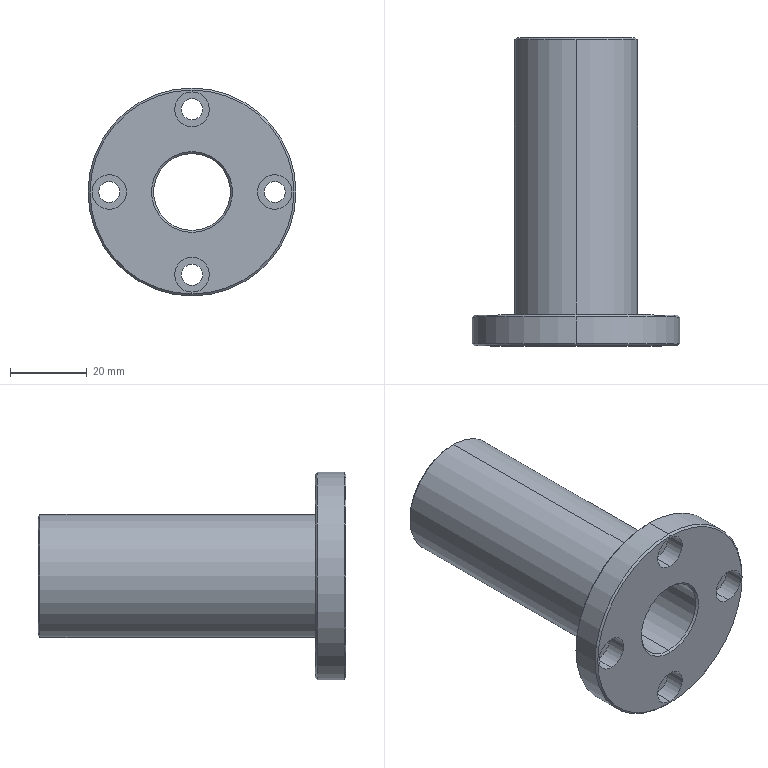Component | SolidWorks | FlangedLinearBearingLMF20L-1 | 1 solid | 39 faces | box 54 x 80 x 54 mm | volume 49451 mm3 | cylinder 22 | cone 10 | plane 7 | commonest cylinder face diameters 9 x8 5.5 x8 32 x2 54 x2 20 x2
STEP:
#1=CARTESIAN_POINT('',(-2.82,-0.6008,10.453));
#2=VERTEX_POINT('',#1);
#3=CARTESIAN_POINT('',(-2.82,-0.6008,10.807));
#4=VERTEX_POINT('',#3);
#5=CARTESIAN_POINT('',(-2.82,-0.6008,10.63));
#6=DIRECTION('',(0.,-1.,-0.));
#7=DIRECTION('',(0.,0.,1.));
#8=AXIS2_PLACEMENT_3D('',#5,#6,#7);
#9=CIRCLE('',#8,0.1772);
#10=EDGE_CURVE('',#2,#4,#9,.T.);
#11=ORIENTED_EDGE('',*,*,#10,.F.);
#12=CARTESIAN_POINT('',(-2.82,-0.8016,10.453));
#13=VERTEX_POINT('',#12);
#14=CARTESIAN_POINT('',(-2.82,-0.8016,10.453));
#15=DIRECTION('',(0.,-1.,-0.));
#16=VECTOR('',#15,39.37);
#17=LINE('',#14,#16);
#18=EDGE_CURVE('',#2,#13,#17,.T.);
#19=ORIENTED_EDGE('',*,*,#18,.T.);
#20=CARTESIAN_POINT('',(-2.82,-0.8016,10.807));
#21=VERTEX_POINT('',#20);
#22=CARTESIAN_POINT('',(-2.82,-0.8016,10.63));
#23=DIRECTION('',(0.,-1.,-0.));
#24=DIRECTION('',(0.,0.,1.));
#25=AXIS2_PLACEMENT_3D('',#22,#23,#24);
#26=CIRCLE('',#25,0.1772);
#27=EDGE_CURVE('',#13,#21,#26,.T.);
#28=ORIENTED_EDGE('',*,*,#27,.T.);
#29=CARTESIAN_POINT('',(-2.82,-0.8016,10.807));
#30=DIRECTION('',(0.,-1.,-0.));
#31=VECTOR('',#30,39.37);
#32=LINE('',#29,#31);
#33=EDGE_CURVE('',#4,#21,#32,.T.);
#34=ORIENTED_EDGE('',*,*,#33,.F.);
#35=EDGE_LOOP('',(#11,#19,#28,#34));
#36=FACE_OUTER_BOUND('',#35,.T.);
#37=CARTESIAN_POINT('',(-2.82,-0.8016,10.63));
#38=DIRECTION('',(0.,-1.,-0.));
#39=DIRECTION('',(0.,0.,1.));
#40=AXIS2_PLACEMENT_3D('',#37,#38,#39);
#41=CYLINDRICAL_SURFACE('',#40,0.1772);
#42=ADVANCED_FACE('',(#36),#41,.F.);
#43=CARTESIAN_POINT('',(-2.82,-0.4866,10.522));
#44=VERTEX_POINT('',#43);
#45=CARTESIAN_POINT('',(-2.82,-0.4866,10.738));
#46=VERTEX_POINT('',#45);
#47=CARTESIAN_POINT('',(-2.82,-0.4866,10.63));
#48=DIRECTION('',(0.,-1.,-0.));
#49=DIRECTION('',(0.,0.,1.));
#50=AXIS2_PLACEMENT_3D('',#47,#48,#49);
#51=CIRCLE('',#50,0.1083);
#52=EDGE_CURVE('',#44,#46,#51,.T.);
#53=ORIENTED_EDGE('',*,*,#52,.F.);
#54=CARTESIAN_POINT('',(-2.82,-0.6008,10.522));
#55=VERTEX_POINT('',#54);
#56=CARTESIAN_POINT('',(-2.82,-0.8016,10.522));
#57=DIRECTION('',(0.,-1.,-0.));
#58=VECTOR('',#57,39.37);
#59=LINE('',#56,#58);
#60=EDGE_CURVE('',#44,#55,#59,.T.);
#61=ORIENTED_EDGE('',*,*,#60,.T.);
#62=CARTESIAN_POINT('',(-2.82,-0.6008,10.738));
#63=VERTEX_POINT('',#62);
#64=CARTESIAN_POINT('',(-2.82,-0.6008,10.63));
#65=DIRECTION('',(0.,-1.,-0.));
#66=DIRECTION('',(0.,0.,1.));
#67=AXIS2_PLACEMENT_3D('',#64,#65,#66);
#68=CIRCLE('',#67,0.1083);
#69=EDGE_CURVE('',#55,#63,#68,.T.);
#70=ORIENTED_EDGE('',*,*,#69,.T.);
#71=CARTESIAN_POINT('',(-2.82,-0.8016,10.738));
#72=DIRECTION('',(0.,-1.,-0.));
#73=VECTOR('',#72,39.37);
#74=LINE('',#71,#73);
#75=EDGE_CURVE('',#46,#63,#74,.T.);
#76=ORIENTED_EDGE('',*,*,#75,.F.);
#77=EDGE_LOOP('',(#53,#61,#70,#76));
#78=FACE_OUTER_BOUND('',#77,.T.);
#79=CARTESIAN_POINT('',(-2.82,-0.8016,10.63));
#80=DIRECTION('',(0.,-1.,-0.));
#81=DIRECTION('',(0.,0.,1.));
#82=AXIS2_PLACEMENT_3D('',#79,#80,#81);
#83=CYLINDRICAL_SURFACE('',#82,0.1083);
#84=ADVANCED_FACE('',(#78),#83,.F.);
#85=CARTESIAN_POINT('',(-1.973,-0.6008,9.606));
#86=VERTEX_POINT('',#85);
#87=CARTESIAN_POINT('',(-1.973,-0.6008,9.961));
#88=VERTEX_POINT('',#87);
#89=CARTESIAN_POINT('',(-1.973,-0.6008,9.783));
#90=DIRECTION('',(0.,-1.,-0.));
#91=DIRECTION('',(0.,0.,1.));
#92=AXIS2_PLACEMENT_3D('',#89,#90,#91);
#93=CIRCLE('',#92,0.1772);
#94=EDGE_CURVE('',#86,#88,#93,.T.);
#95=ORIENTED_EDGE('',*,*,#94,.F.);
#96=CARTESIAN_POINT('',(-1.973,-0.8016,9.606));
#97=VERTEX_POINT('',#96);
#98=CARTESIAN_POINT('',(-1.973,-0.8016,9.606));
#99=DIRECTION('',(0.,-1.,-0.));
#100=VECTOR('',#99,39.37);
#101=LINE('',#98,#100);
#102=EDGE_CURVE('',#86,#97,#101,.T.);
#103=ORIENTED_EDGE('',*,*,#102,.T.);
#104=CARTESIAN_POINT('',(-1.973,-0.8016,9.961));
#105=VERTEX_POINT('',#104);
#106=CARTESIAN_POINT('',(-1.973,-0.8016,9.783));
#107=DIRECTION('',(0.,-1.,-0.));
#108=DIRECTION('',(0.,0.,1.));
#109=AXIS2_PLACEMENT_3D('',#106,#107,#108);
#110=CIRCLE('',#109,0.1772);
#111=EDGE_CURVE('',#97,#105,#110,.T.);
#112=ORIENTED_EDGE('',*,*,#111,.T.);
#113=CARTESIAN_POINT('',(-1.973,-0.8016,9.961));
#114=DIRECTION('',(0.,-1.,-0.));
#115=VECTOR('',#114,39.37);
#116=LINE('',#113,#115);
#117=EDGE_CURVE('',#88,#105,#116,.T.);
#118=ORIENTED_EDGE('',*,*,#117,.F.);
#119=EDGE_LOOP('',(#95,#103,#112,#118));
#120=FACE_OUTER_BOUND('',#119,.T.);
#121=CARTESIAN_POINT('',(-1.973,-0.8016,9.783));
#122=DIRECTION('',(0.,-1.,-0.));
#123=DIRECTION('',(0.,0.,1.));
#124=AXIS2_PLACEMENT_3D('',#121,#122,#123);
#125=CYLINDRICAL_SURFACE('',#124,0.1772);
#126=ADVANCED_FACE('',(#120),#125,.F.);
#127=CARTESIAN_POINT('',(-1.973,-0.4866,9.675));
#128=VERTEX_POINT('',#127);
#129=CARTESIAN_POINT('',(-1.973,-0.4866,9.892));
#130=VERTEX_POINT('',#129);
#131=CARTESIAN_POINT('',(-1.973,-0.4866,9.783));
#132=DIRECTION('',(0.,-1.,-0.));
#133=DIRECTION('',(0.,0.,1.));
#134=AXIS2_PLACEMENT_3D('',#131,#132,#133);
#135=CIRCLE('',#134,0.1083);
#136=EDGE_CURVE('',#128,#130,#135,.T.);
#137=ORIENTED_EDGE('',*,*,#136,.F.);
#138=CARTESIAN_POINT('',(-1.973,-0.6008,9.675));
#139=VERTEX_POINT('',#138);
#140=CARTESIAN_POINT('',(-1.973,-0.8016,9.675));
#141=DIRECTION('',(0.,-1.,-0.));
#142=VECTOR('',#141,39.37);
#143=LINE('',#140,#142);
#144=EDGE_CURVE('',#128,#139,#143,.T.);
#145=ORIENTED_EDGE('',*,*,#144,.T.);
#146=CARTESIAN_POINT('',(-1.973,-0.6008,9.892));
#147=VERTEX_POINT('',#146);
#148=CARTESIAN_POINT('',(-1.973,-0.6008,9.783));
#149=DIRECTION('',(0.,-1.,-0.));
#150=DIRECTION('',(0.,0.,1.));
#151=AXIS2_PLACEMENT_3D('',#148,#149,#150);
#152=CIRCLE('',#151,0.1083);
#153=EDGE_CURVE('',#139,#147,#152,.T.);
#154=ORIENTED_EDGE('',*,*,#153,.T.);
#155=CARTESIAN_POINT('',(-1.973,-0.8016,9.892));
#156=DIRECTION('',(0.,-1.,-0.));
#157=VECTOR('',#156,39.37);
#158=LINE('',#155,#157);
#159=EDGE_CURVE('',#130,#147,#158,.T.);
#160=ORIENTED_EDGE('',*,*,#159,.F.);
#161=EDGE_LOOP('',(#137,#145,#154,#160));
#162=FACE_OUTER_BOUND('',#161,.T.);
#163=CARTESIAN_POINT('',(-1.973,-0.8016,9.783));
#164=DIRECTION('',(0.,-1.,-0.));
#165=DIRECTION('',(0.,0.,1.));
#166=AXIS2_PLACEMENT_3D('',#163,#164,#165);
#167=CYLINDRICAL_SURFACE('',#166,0.1083);
#168=ADVANCED_FACE('',(#162),#167,.F.);
#169=CARTESIAN_POINT('',(-1.973,-0.6008,11.299));
#170=VERTEX_POINT('',#169);
#171=CARTESIAN_POINT('',(-1.973,-0.6008,11.654));
#172=VERTEX_POINT('',#171);
#173=CARTESIAN_POINT('',(-1.973,-0.6008,11.476));
#174=DIRECTION('',(0.,-1.,-0.));
#175=DIRECTION('',(0.,0.,1.));
#176=AXIS2_PLACEMENT_3D('',#173,#174,#175);
#177=CIRCLE('',#176,0.1772);
#178=EDGE_CURVE('',#170,#172,#177,.T.);
#179=ORIENTED_EDGE('',*,*,#178,.F.);
#180=CARTESIAN_POINT('',(-1.973,-0.8016,11.299));
#181=VERTEX_POINT('',#180);
#182=CARTESIAN_POINT('',(-1.973,-0.8016,11.299));
#183=DIRECTION('',(0.,-1.,-0.));
#184=VECTOR('',#183,39.37);
#185=LINE('',#182,#184);
#186=EDGE_CURVE('',#170,#181,#185,.T.);
#187=ORIENTED_EDGE('',*,*,#186,.T.);
#188=CARTESIAN_POINT('',(-1.973,-0.8016,11.654));
#189=VERTEX_POINT('',#188);
#190=CARTESIAN_POINT('',(-1.973,-0.8016,11.476));
#191=DIRECTION('',(0.,-1.,-0.));
#192=DIRECTION('',(0.,0.,1.));
#193=AXIS2_PLACEMENT_3D('',#190,#191,#192);
#194=CIRCLE('',#193,0.1772);
#195=EDGE_CURVE('',#181,#189,#194,.T.);
#196=ORIENTED_EDGE('',*,*,#195,.T.);
#197=CARTESIAN_POINT('',(-1.973,-0.8016,11.654));
#198=DIRECTION('',(0.,-1.,-0.));
#199=VECTOR('',#198,39.37);
#200=LINE('',#197,#199);
#201=EDGE_CURVE('',#172,#189,#200,.T.);
#202=ORIENTED_EDGE('',*,*,#201,.F.);
#203=EDGE_LOOP('',(#179,#187,#196,#202));
#204=FACE_OUTER_BOUND('',#203,.T.);
#205=CARTESIAN_POINT('',(-1.973,-0.8016,11.476));
#206=DIRECTION('',(0.,-1.,-0.));
#207=DIRECTION('',(0.,0.,1.));
#208=AXIS2_PLACEMENT_3D('',#205,#206,#207);
#209=CYLINDRICAL_SURFACE('',#208,0.1772);
#210=ADVANCED_FACE('',(#204),#209,.F.);
#211=CARTESIAN_POINT('',(-1.973,-0.4866,11.368));
#212=VERTEX_POINT('',#211);
#213=CARTESIAN_POINT('',(-1.973,-0.4866,11.585));
#214=VERTEX_POINT('',#213);
#215=CARTESIAN_POINT('',(-1.973,-0.4866,11.476));
#216=DIRECTION('',(0.,-1.,-0.));
#217=DIRECTION('',(0.,0.,1.));
#218=AXIS2_PLACEMENT_3D('',#215,#216,#217);
#219=CIRCLE('',#218,0.1083);
#220=EDGE_CURVE('',#212,#214,#219,.T.);
#221=ORIENTED_EDGE('',*,*,#220,.F.);
#222=CARTESIAN_POINT('',(-1.973,-0.6008,11.368));
#223=VERTEX_POINT('',#222);
#224=CARTESIAN_POINT('',(-1.973,-0.8016,11.368));
#225=DIRECTION('',(0.,-1.,-0.));
#226=VECTOR('',#225,39.37);
#227=LINE('',#224,#226);
#228=EDGE_CURVE('',#212,#223,#227,.T.);
#229=ORIENTED_EDGE('',*,*,#228,.T.);
#230=CARTESIAN_POINT('',(-1.973,-0.6008,11.585));
#231=VERTEX_POINT('',#230);
#232=CARTESIAN_POINT('',(-1.973,-0.6008,11.476));
#233=DIRECTION('',(0.,-1.,-0.));
#234=DIRECTION('',(0.,0.,1.));
#235=AXIS2_PLACEMENT_3D('',#232,#233,#234);
#236=CIRCLE('',#235,0.1083);
#237=EDGE_CURVE('',#223,#231,#236,.T.);
#238=ORIENTED_EDGE('',*,*,#237,.T.);
#239=CARTESIAN_POINT('',(-1.973,-0.8016,11.585));
#240=DIRECTION('',(0.,-1.,-0.));
#241=VECTOR('',#240,39.37);
#242=LINE('',#239,#241);
#243=EDGE_CURVE('',#214,#231,#242,.T.);
#244=ORIENTED_EDGE('',*,*,#243,.F.);
#245=EDGE_LOOP('',(#221,#229,#238,#244));
#246=FACE_OUTER_BOUND('',#245,.T.);
#247=CARTESIAN_POINT('',(-1.973,-0.8016,11.476));
#248=DIRECTION('',(0.,-1.,-0.));
#249=DIRECTION('',(0.,0.,1.));
#250=AXIS2_PLACEMENT_3D('',#247,#248,#249);
#251=CYLINDRICAL_SURFACE('',#250,0.1083);
#252=ADVANCED_FACE('',(#246),#251,.F.);
#253=CARTESIAN_POINT('',(-1.127,-0.6008,10.453));
#254=VERTEX_POINT('',#253);
#255=CARTESIAN_POINT('',(-1.127,-0.6008,10.807));
#256=VERTEX_POINT('',#255);
#257=CARTESIAN_POINT('',(-1.127,-0.6008,10.63));
#258=DIRECTION('',(0.,-1.,-0.));
#259=DIRECTION('',(0.,0.,1.));
#260=AXIS2_PLACEMENT_3D('',#257,#258,#259);
#261=CIRCLE('',#260,0.1772);
#262=EDGE_CURVE('',#254,#256,#261,.T.);
#263=ORIENTED_EDGE('',*,*,#262,.F.);
#264=CARTESIAN_POINT('',(-1.127,-0.8016,10.453));
#265=VERTEX_POINT('',#264);
#266=CARTESIAN_POINT('',(-1.127,-0.8016,10.453));
#267=DIRECTION('',(0.,-1.,-0.));
#268=VECTOR('',#267,39.37);
#269=LINE('',#266,#268);
#270=EDGE_CURVE('',#254,#265,#269,.T.);
#271=ORIENTED_EDGE('',*,*,#270,.T.);
#272=CARTESIAN_POINT('',(-1.127,-0.8016,10.807));
#273=VERTEX_POINT('',#272);
#274=CARTESIAN_POINT('',(-1.127,-0.8016,10.63));
#275=DIRECTION('',(0.,-1.,-0.));
#276=DIRECTION('',(0.,0.,1.));
#277=AXIS2_PLACEMENT_3D('',#274,#275,#276);
#278=CIRCLE('',#277,0.1772);
#279=EDGE_CURVE('',#265,#273,#278,.T.);
#280=ORIENTED_EDGE('',*,*,#279,.T.);
#281=CARTESIAN_POINT('',(-1.127,-0.8016,10.807));
#282=DIRECTION('',(0.,-1.,-0.));
#283=VECTOR('',#282,39.37);
#284=LINE('',#281,#283);
#285=EDGE_CURVE('',#256,#273,#284,.T.);
#286=ORIENTED_EDGE('',*,*,#285,.F.);
#287=EDGE_LOOP('',(#263,#271,#280,#286));
#288=FACE_OUTER_BOUND('',#287,.T.);
#289=CARTESIAN_POINT('',(-1.127,-0.8016,10.63));
#290=DIRECTION('',(0.,-1.,-0.));
#291=DIRECTION('',(0.,0.,1.));
#292=AXIS2_PLACEMENT_3D('',#289,#290,#291);
#293=CYLINDRICAL_SURFACE('',#292,0.1772);
#294=ADVANCED_FACE('',(#288),#293,.F.);
#295=CARTESIAN_POINT('',(-1.127,-0.4866,10.522));
#296=VERTEX_POINT('',#295);
#297=CARTESIAN_POINT('',(-1.127,-0.4866,10.738));
#298=VERTEX_POINT('',#297);
#299=CARTESIAN_POINT('',(-1.127,-0.4866,10.63));
#300=DIRECTION('',(0.,-1.,-0.));
#301=DIRECTION('',(0.,0.,1.));
#302=AXIS2_PLACEMENT_3D('',#299,#300,#301);
#303=CIRCLE('',#302,0.1083);
#304=EDGE_CURVE('',#296,#298,#303,.T.);
#305=ORIENTED_EDGE('',*,*,#304,.F.);
#306=CARTESIAN_POINT('',(-1.127,-0.6008,10.522));
#307=VERTEX_POINT('',#306);
#308=CARTESIAN_POINT('',(-1.127,-0.8016,10.522));
#309=DIRECTION('',(0.,-1.,-0.));
#310=VECTOR('',#309,39.37);
#311=LINE('',#308,#310);
#312=EDGE_CURVE('',#296,#307,#311,.T.);
#313=ORIENTED_EDGE('',*,*,#312,.T.);
#314=CARTESIAN_POINT('',(-1.127,-0.6008,10.738));
#315=VERTEX_POINT('',#314);
#316=CARTESIAN_POINT('',(-1.127,-0.6008,10.63));
#317=DIRECTION('',(0.,-1.,-0.));
#318=DIRECTION('',(0.,0.,1.));
#319=AXIS2_PLACEMENT_3D('',#316,#317,#318);
#320=CIRCLE('',#319,0.1083);
#321=EDGE_CURVE('',#307,#315,#320,.T.);
#322=ORIENTED_EDGE('',*,*,#321,.T.);
#323=CARTESIAN_POINT('',(-1.127,-0.8016,10.738));
#324=DIRECTION('',(0.,-1.,-0.));
#325=VECTOR('',#324,39.37);
#326=LINE('',#323,#325);
#327=EDGE_CURVE('',#298,#315,#326,.T.);
#328=ORIENTED_EDGE('',*,*,#327,.F.);
#329=EDGE_LOOP('',(#305,#313,#322,#328));
#330=FACE_OUTER_BOUND('',#329,.T.);
#331=CARTESIAN_POINT('',(-1.127,-0.8016,10.63));
#332=DIRECTION('',(0.,-1.,-0.));
#333=DIRECTION('',(0.,0.,1.));
#334=AXIS2_PLACEMENT_3D('',#331,#332,#333);
#335=CYLINDRICAL_SURFACE('',#334,0.1083);
#336=ADVANCED_FACE('',(#330),#335,.F.);
#337=CARTESIAN_POINT('',(-1.973,-0.8016,11.673));
#338=VERTEX_POINT('',#337);
#339=CARTESIAN_POINT('',(-1.973,-0.8016,9.587));
#340=VERTEX_POINT('',#339);
#341=CARTESIAN_POINT('',(-1.973,-0.8016,10.63));
#342=DIRECTION('',(0.,-1.,-0.));
#343=DIRECTION('',(-0.,0.,-1.));
#344=AXIS2_PLACEMENT_3D('',#341,#342,#343);
#345=CIRCLE('',#344,1.043);
#346=EDGE_CURVE('',#338,#340,#345,.T.);
#347=ORIENTED_EDGE('',*,*,#346,.F.);
#348=CARTESIAN_POINT('',(-1.973,-0.7819,11.693));
#349=VERTEX_POINT('',#348);
#350=CARTESIAN_POINT('',(-1.973,-0.8016,11.673));
#351=DIRECTION('',(0.,0.7071,0.7071));
#352=VECTOR('',#351,39.37);
#353=LINE('',#350,#352);
#354=EDGE_CURVE('',#338,#349,#353,.T.);
#355=ORIENTED_EDGE('',*,*,#354,.T.);
#356=CARTESIAN_POINT('',(-1.973,-0.7819,9.567));
#357=VERTEX_POINT('',#356);
#358=CARTESIAN_POINT('',(-1.973,-0.7819,10.63));
#359=DIRECTION('',(-0.,1.,0.));
#360=DIRECTION('',(-0.,0.,-1.));
#361=AXIS2_PLACEMENT_3D('',#358,#359,#360);
#362=CIRCLE('',#361,1.063);
#363=EDGE_CURVE('',#357,#349,#362,.T.);
#364=ORIENTED_EDGE('',*,*,#363,.F.);
#365=CARTESIAN_POINT('',(-1.973,-0.8016,9.587));
#366=DIRECTION('',(-0.,0.7071,-0.7071));
#367=VECTOR('',#366,39.37);
#368=LINE('',#365,#367);
#369=EDGE_CURVE('',#340,#357,#368,.T.);
#370=ORIENTED_EDGE('',*,*,#369,.F.);
#371=EDGE_LOOP('',(#347,#355,#364,#370));
#372=FACE_OUTER_BOUND('',#371,.T.);
#373=CARTESIAN_POINT('',(-1.973,-0.8016,10.63));
#374=DIRECTION('',(-0.,1.,0.));
#375=DIRECTION('',(-0.,0.,-1.));
#376=AXIS2_PLACEMENT_3D('',#373,#374,#375);
#377=CONICAL_SURFACE('',#376,1.043,0.7854);
#378=ADVANCED_FACE('',(#372),#377,.T.);
#379=CARTESIAN_POINT('',(-1.973,-0.4866,9.587));
#380=VERTEX_POINT('',#379);
#381=CARTESIAN_POINT('',(-1.973,-0.4866,11.673));
#382=VERTEX_POINT('',#381);
#383=CARTESIAN_POINT('',(-1.973,-0.4866,10.63));
#384=DIRECTION('',(-0.,1.,0.));
#385=DIRECTION('',(0.,-0.,1.));
#386=AXIS2_PLACEMENT_3D('',#383,#384,#385);
#387=CIRCLE('',#386,1.043);
#388=EDGE_CURVE('',#380,#382,#387,.T.);
#389=ORIENTED_EDGE('',*,*,#388,.F.);
#390=CARTESIAN_POINT('',(-1.973,-0.5063,9.567));
#391=VERTEX_POINT('',#390);
#392=CARTESIAN_POINT('',(-1.973,-0.5063,9.567));
#393=DIRECTION('',(-0.,-0.7071,-0.7071));
#394=VECTOR('',#393,39.37);
#395=LINE('',#392,#394);
#396=EDGE_CURVE('',#380,#391,#395,.T.);
#397=ORIENTED_EDGE('',*,*,#396,.T.);
#398=CARTESIAN_POINT('',(-1.973,-0.5063,11.693));
#399=VERTEX_POINT('',#398);
#400=CARTESIAN_POINT('',(-1.973,-0.5063,10.63));
#401=DIRECTION('',(0.,-1.,-0.));
#402=DIRECTION('',(0.,-0.,1.));
#403=AXIS2_PLACEMENT_3D('',#400,#401,#402);
#404=CIRCLE('',#403,1.063);
#405=EDGE_CURVE('',#399,#391,#404,.T.);
#406=ORIENTED_EDGE('',*,*,#405,.F.);
#407=CARTESIAN_POINT('',(-1.973,-0.5063,11.693));
#408=DIRECTION('',(0.,-0.7071,0.7071));
#409=VECTOR('',#408,39.37);
#410=LINE('',#407,#409);
#411=EDGE_CURVE('',#382,#399,#410,.T.);
#412=ORIENTED_EDGE('',*,*,#411,.F.);
#413=EDGE_LOOP('',(#389,#397,#406,#412));
#414=FACE_OUTER_BOUND('',#413,.T.);
#415=CARTESIAN_POINT('',(-1.973,-0.5063,10.63));
#416=DIRECTION('',(0.,-1.,-0.));
#417=DIRECTION('',(0.,-0.,1.));
#418=AXIS2_PLACEMENT_3D('',#415,#416,#417);
#419=CONICAL_SURFACE('',#418,1.063,0.7854);
#420=ADVANCED_FACE('',(#414),#419,.T.);
#421=CARTESIAN_POINT('',(-1.973,-0.7819,10.236));
#422=VERTEX_POINT('',#421);
#423=CARTESIAN_POINT('',(-1.973,-0.7819,11.024));
#424=VERTEX_POINT('',#423);
#425=CARTESIAN_POINT('',(-1.973,-0.7819,10.63));
#426=DIRECTION('',(0.,-1.,-0.));
#427=DIRECTION('',(-0.,0.,-1.));
#428=AXIS2_PLACEMENT_3D('',#425,#426,#427);
#429=CIRCLE('',#428,0.3937);
#430=EDGE_CURVE('',#422,#424,#429,.T.);
#431=ORIENTED_EDGE('',*,*,#430,.F.);
#432=CARTESIAN_POINT('',(-1.973,-0.8016,10.217));
#433=VERTEX_POINT('',#432);
#434=CARTESIAN_POINT('',(-1.973,-0.7819,10.236));
#435=DIRECTION('',(-0.,-0.7071,-0.7071));
#436=VECTOR('',#435,39.37);
#437=LINE('',#434,#436);
#438=EDGE_CURVE('',#422,#433,#437,.T.);
#439=ORIENTED_EDGE('',*,*,#438,.T.);
#440=CARTESIAN_POINT('',(-1.973,-0.8016,11.043));
#441=VERTEX_POINT('',#440);
#442=CARTESIAN_POINT('',(-1.973,-0.8016,10.63));
#443=DIRECTION('',(-0.,1.,0.));
#444=DIRECTION('',(-0.,0.,-1.));
#445=AXIS2_PLACEMENT_3D('',#442,#443,#444);
#446=CIRCLE('',#445,0.4134);
#447=EDGE_CURVE('',#441,#433,#446,.T.);
#448=ORIENTED_EDGE('',*,*,#447,.F.);
#449=CARTESIAN_POINT('',(-1.973,-0.7819,11.024));
#450=DIRECTION('',(0.,-0.7071,0.7071));
#451=VECTOR('',#450,39.37);
#452=LINE('',#449,#451);
#453=EDGE_CURVE('',#424,#441,#452,.T.);
#454=ORIENTED_EDGE('',*,*,#453,.F.);
#455=EDGE_LOOP('',(#431,#439,#448,#454));
#456=FACE_OUTER_BOUND('',#455,.T.);
#457=CARTESIAN_POINT('',(-1.973,-0.7819,10.63));
#458=DIRECTION('',(0.,-1.,-0.));
#459=DIRECTION('',(0.,0.,1.));
#460=AXIS2_PLACEMENT_3D('',#457,#458,#459);
#461=CONICAL_SURFACE('',#460,0.3937,0.7854);
#462=ADVANCED_FACE('',(#456),#461,.F.);
#463=CARTESIAN_POINT('',(-1.973,2.348,10.02));
#464=VERTEX_POINT('',#463);
#465=CARTESIAN_POINT('',(-1.973,2.348,11.24));
#466=VERTEX_POINT('',#465);
#467=CARTESIAN_POINT('',(-1.973,2.348,10.63));
#468=DIRECTION('',(-0.,1.,0.));
#469=DIRECTION('',(0.,0.,1.));
#470=AXIS2_PLACEMENT_3D('',#467,#468,#469);
#471=CIRCLE('',#470,0.6102);
#472=EDGE_CURVE('',#464,#466,#471,.T.);
#473=ORIENTED_EDGE('',*,*,#472,.F.);
#474=CARTESIAN_POINT('',(-1.973,2.328,10.));
#475=VERTEX_POINT('',#474);
#476=CARTESIAN_POINT('',(-1.973,2.328,10.));
#477=DIRECTION('',(-0.,-0.7071,-0.7071));
#478=VECTOR('',#477,39.37);
#479=LINE('',#476,#478);
#480=EDGE_CURVE('',#464,#475,#479,.T.);
#481=ORIENTED_EDGE('',*,*,#480,.T.);
#482=CARTESIAN_POINT('',(-1.973,2.328,11.26));
#483=VERTEX_POINT('',#482);
#484=CARTESIAN_POINT('',(-1.973,2.328,10.63));
#485=DIRECTION('',(0.,-1.,-0.));
#486=DIRECTION('',(0.,0.,1.));
#487=AXIS2_PLACEMENT_3D('',#484,#485,#486);
#488=CIRCLE('',#487,0.6299);
#489=EDGE_CURVE('',#483,#475,#488,.T.);
#490=ORIENTED_EDGE('',*,*,#489,.F.);
#491=CARTESIAN_POINT('',(-1.973,2.328,11.26));
#492=DIRECTION('',(0.,-0.7071,0.7071));
#493=VECTOR('',#492,39.37);
#494=LINE('',#491,#493);
#495=EDGE_CURVE('',#466,#483,#494,.T.);
#496=ORIENTED_EDGE('',*,*,#495,.F.);
#497=EDGE_LOOP('',(#473,#481,#490,#496));
#498=FACE_OUTER_BOUND('',#497,.T.);
#499=CARTESIAN_POINT('',(-1.973,2.328,10.63));
#500=DIRECTION('',(0.,-1.,-0.));
#501=DIRECTION('',(0.,0.,1.));
#502=AXIS2_PLACEMENT_3D('',#499,#500,#501);
#503=CONICAL_SURFACE('',#502,0.6299,0.7854);
#504=ADVANCED_FACE('',(#498),#503,.T.);
#505=CARTESIAN_POINT('',(-1.973,2.328,11.024));
#506=VERTEX_POINT('',#505);
#507=CARTESIAN_POINT('',(-1.973,2.328,10.236));
#508=VERTEX_POINT('',#507);
#509=CARTESIAN_POINT('',(-1.973,2.328,10.63));
#510=DIRECTION('',(-0.,1.,0.));
#511=DIRECTION('',(0.,0.,1.));
#512=AXIS2_PLACEMENT_3D('',#509,#510,#511);
#513=CIRCLE('',#512,0.3937);
#514=EDGE_CURVE('',#506,#508,#513,.T.);
#515=ORIENTED_EDGE('',*,*,#514,.F.);
#516=CARTESIAN_POINT('',(-1.973,2.348,11.043));
#517=VERTEX_POINT('',#516);
#518=CARTESIAN_POINT('',(-1.973,2.348,11.043));
#519=DIRECTION('',(0.,0.7071,0.7071));
#520=VECTOR('',#519,39.37);
#521=LINE('',#518,#520);
#522=EDGE_CURVE('',#506,#517,#521,.T.);
#523=ORIENTED_EDGE('',*,*,#522,.T.);
#524=CARTESIAN_POINT('',(-1.973,2.348,10.217));
#525=VERTEX_POINT('',#524);
#526=CARTESIAN_POINT('',(-1.973,2.348,10.63));
#527=DIRECTION('',(0.,-1.,-0.));
#528=DIRECTION('',(0.,0.,1.));
#529=AXIS2_PLACEMENT_3D('',#526,#527,#528);
#530=CIRCLE('',#529,0.4134);
#531=EDGE_CURVE('',#525,#517,#530,.T.);
#532=ORIENTED_EDGE('',*,*,#531,.F.);
#533=CARTESIAN_POINT('',(-1.973,2.348,10.217));
#534=DIRECTION('',(-0.,0.7071,-0.7071));
#535=VECTOR('',#534,39.37);
#536=LINE('',#533,#535);
#537=EDGE_CURVE('',#508,#525,#536,.T.);
#538=ORIENTED_EDGE('',*,*,#537,.F.);
#539=EDGE_LOOP('',(#515,#523,#532,#538));
#540=FACE_OUTER_BOUND('',#539,.T.);
#541=CARTESIAN_POINT('',(-1.973,2.348,10.63));
#542=DIRECTION('',(-0.,1.,0.));
#543=DIRECTION('',(-0.,0.,-1.));
#544=AXIS2_PLACEMENT_3D('',#541,#542,#543);
#545=CONICAL_SURFACE('',#544,0.4134,0.7854);
#546=ADVANCED_FACE('',(#540),#545,.F.);
#547=ORIENTED_EDGE('',*,*,#489,.T.);
#548=CARTESIAN_POINT('',(-1.973,-0.4866,10.));
#549=VERTEX_POINT('',#548);
#550=CARTESIAN_POINT('',(-1.973,-0.8016,10.));
#551=DIRECTION('',(0.,-1.,-0.));
#552=VECTOR('',#551,39.37);
#553=LINE('',#550,#552);
#554=EDGE_CURVE('',#475,#549,#553,.T.);
#555=ORIENTED_EDGE('',*,*,#554,.T.);
#556=CARTESIAN_POINT('',(-1.973,-0.4866,11.26));
#557=VERTEX_POINT('',#556);
#558=CARTESIAN_POINT('',(-1.973,-0.4866,10.63));
#559=DIRECTION('',(0.,-1.,-0.));
#560=DIRECTION('',(0.,-0.,1.));
#561=AXIS2_PLACEMENT_3D('',#558,#559,#560);
#562=CIRCLE('',#561,0.6299);
#563=EDGE_CURVE('',#557,#549,#562,.T.);
#564=ORIENTED_EDGE('',*,*,#563,.F.);
#565=CARTESIAN_POINT('',(-1.973,-0.8016,11.26));
#566=DIRECTION('',(0.,-1.,-0.));
#567=VECTOR('',#566,39.37);
#568=LINE('',#565,#567);
#569=EDGE_CURVE('',#483,#557,#568,.T.);
#570=ORIENTED_EDGE('',*,*,#569,.F.);
#571=EDGE_LOOP('',(#547,#555,#564,#570));
#572=FACE_OUTER_BOUND('',#571,.T.);
#573=CARTESIAN_POINT('',(-1.973,-0.8016,10.63));
#574=DIRECTION('',(0.,-1.,-0.));
#575=DIRECTION('',(0.,0.,1.));
#576=AXIS2_PLACEMENT_3D('',#573,#574,#575);
#577=CYLINDRICAL_SURFACE('',#576,0.6299);
#578=ADVANCED_FACE('',(#572),#577,.T.);
#579=ORIENTED_EDGE('',*,*,#405,.T.);
#580=CARTESIAN_POINT('',(-1.973,-0.8016,9.567));
#581=DIRECTION('',(0.,-1.,-0.));
#582=VECTOR('',#581,39.37);
#583=LINE('',#580,#582);
#584=EDGE_CURVE('',#391,#357,#583,.T.);
#585=ORIENTED_EDGE('',*,*,#584,.T.);
#586=ORIENTED_EDGE('',*,*,#363,.T.);
#587=CARTESIAN_POINT('',(-1.973,-0.8016,11.693));
#588=DIRECTION('',(0.,-1.,-0.));
#589=VECTOR('',#588,39.37);
#590=LINE('',#587,#589);
#591=EDGE_CURVE('',#399,#349,#590,.T.);
#592=ORIENTED_EDGE('',*,*,#591,.F.);
#593=EDGE_LOOP('',(#579,#585,#586,#592));
#594=FACE_OUTER_BOUND('',#593,.T.);
#595=CARTESIAN_POINT('',(-1.973,-0.8016,10.63));
#596=DIRECTION('',(0.,-1.,-0.));
#597=DIRECTION('',(0.,-0.,1.));
#598=AXIS2_PLACEMENT_3D('',#595,#596,#597);
#599=CYLINDRICAL_SURFACE('',#598,1.063);
#600=ADVANCED_FACE('',(#594),#599,.T.);
#601=ORIENTED_EDGE('',*,*,#514,.T.);
#602=CARTESIAN_POINT('',(-1.973,-0.8016,10.236));
#603=DIRECTION('',(0.,-1.,-0.));
#604=VECTOR('',#603,39.37);
#605=LINE('',#602,#604);
#606=EDGE_CURVE('',#508,#422,#605,.T.);
#607=ORIENTED_EDGE('',*,*,#606,.T.);
#608=ORIENTED_EDGE('',*,*,#430,.T.);
#609=CARTESIAN_POINT('',(-1.973,-0.8016,11.024));
#610=DIRECTION('',(0.,-1.,-0.));
#611=VECTOR('',#610,39.37);
#612=LINE('',#609,#611);
#613=EDGE_CURVE('',#506,#424,#612,.T.);
#614=ORIENTED_EDGE('',*,*,#613,.F.);
#615=EDGE_LOOP('',(#601,#607,#608,#614));
#616=FACE_OUTER_BOUND('',#615,.T.);
#617=CARTESIAN_POINT('',(-1.973,-0.8016,10.63));
#618=DIRECTION('',(0.,-1.,-0.));
#619=DIRECTION('',(0.,0.,1.));
#620=AXIS2_PLACEMENT_3D('',#617,#618,#619);
#621=CYLINDRICAL_SURFACE('',#620,0.3937);
#622=ADVANCED_FACE('',(#616),#621,.F.);
#623=ORIENTED_EDGE('',*,*,#606,.F.);
#624=CARTESIAN_POINT('',(-1.973,2.328,10.63));
#625=DIRECTION('',(-0.,1.,0.));
#626=DIRECTION('',(0.,0.,1.));
#627=AXIS2_PLACEMENT_3D('',#624,#625,#626);
#628=CIRCLE('',#627,0.3937);
#629=EDGE_CURVE('',#508,#506,#628,.T.);
#630=ORIENTED_EDGE('',*,*,#629,.T.);
#631=ORIENTED_EDGE('',*,*,#613,.T.);
#632=CARTESIAN_POINT('',(-1.973,-0.7819,10.63));
#633=DIRECTION('',(0.,-1.,-0.));
#634=DIRECTION('',(0.,0.,-1.));
#635=AXIS2_PLACEMENT_3D('',#632,#633,#634);
#636=CIRCLE('',#635,0.3937);
#637=EDGE_CURVE('',#424,#422,#636,.T.);
#638=ORIENTED_EDGE('',*,*,#637,.T.);
#639=EDGE_LOOP('',(#623,#630,#631,#638));
#640=FACE_OUTER_BOUND('',#639,.T.);
#641=CARTESIAN_POINT('',(-1.973,-0.8016,10.63));
#642=DIRECTION('',(0.,-1.,-0.));
#643=DIRECTION('',(0.,0.,1.));
#644=AXIS2_PLACEMENT_3D('',#641,#642,#643);
#645=CYLINDRICAL_SURFACE('',#644,0.3937);
#646=ADVANCED_FACE('',(#640),#645,.F.);
#647=CARTESIAN_POINT('',(-2.82,-0.8016,10.63));
#648=DIRECTION('',(0.,-1.,-0.));
#649=DIRECTION('',(0.,0.,1.));
#650=AXIS2_PLACEMENT_3D('',#647,#648,#649);
#651=CIRCLE('',#650,0.1772);
#652=EDGE_CURVE('',#21,#13,#651,.T.);
#653=ORIENTED_EDGE('',*,*,#652,.F.);
#654=ORIENTED_EDGE('',*,*,#27,.F.);
#655=EDGE_LOOP('',(#653,#654));
#656=FACE_BOUND('',#655,.T.);
#657=CARTESIAN_POINT('',(-1.973,-0.8016,9.783));
#658=DIRECTION('',(0.,-1.,-0.));
#659=DIRECTION('',(0.,0.,1.));
#660=AXIS2_PLACEMENT_3D('',#657,#658,#659);
#661=CIRCLE('',#660,0.1772);
#662=EDGE_CURVE('',#105,#97,#661,.T.);
#663=ORIENTED_EDGE('',*,*,#662,.F.);
#664=ORIENTED_EDGE('',*,*,#111,.F.);
#665=EDGE_LOOP('',(#663,#664));
#666=FACE_BOUND('',#665,.T.);
#667=CARTESIAN_POINT('',(-1.973,-0.8016,11.476));
#668=DIRECTION('',(0.,-1.,-0.));
#669=DIRECTION('',(0.,0.,1.));
#670=AXIS2_PLACEMENT_3D('',#667,#668,#669);
#671=CIRCLE('',#670,0.1772);
#672=EDGE_CURVE('',#189,#181,#671,.T.);
#673=ORIENTED_EDGE('',*,*,#672,.F.);
#674=ORIENTED_EDGE('',*,*,#195,.F.);
#675=EDGE_LOOP('',(#673,#674));
#676=FACE_BOUND('',#675,.T.);
#677=CARTESIAN_POINT('',(-1.127,-0.8016,10.63));
#678=DIRECTION('',(0.,-1.,-0.));
#679=DIRECTION('',(0.,0.,1.));
#680=AXIS2_PLACEMENT_3D('',#677,#678,#679);
#681=CIRCLE('',#680,0.1772);
#682=EDGE_CURVE('',#273,#265,#681,.T.);
#683=ORIENTED_EDGE('',*,*,#682,.F.);
#684=ORIENTED_EDGE('',*,*,#279,.F.);
#685=EDGE_LOOP('',(#683,#684));
#686=FACE_BOUND('',#685,.T.);
#687=ORIENTED_EDGE('',*,*,#447,.T.);
#688=CARTESIAN_POINT('',(-1.973,-0.8016,10.63));
#689=DIRECTION('',(-0.,1.,0.));
#690=DIRECTION('',(-0.,0.,-1.));
#691=AXIS2_PLACEMENT_3D('',#688,#689,#690);
#692=CIRCLE('',#691,0.4134);
#693=EDGE_CURVE('',#433,#441,#692,.T.);
#694=ORIENTED_EDGE('',*,*,#693,.T.);
#695=EDGE_LOOP('',(#687,#694));
#696=FACE_BOUND('',#695,.T.);
#697=CARTESIAN_POINT('',(-1.973,-0.8016,10.63));
#698=DIRECTION('',(0.,-1.,-0.));
#699=DIRECTION('',(-0.,0.,-1.));
#700=AXIS2_PLACEMENT_3D('',#697,#698,#699);
#701=CIRCLE('',#700,1.043);
#702=EDGE_CURVE('',#340,#338,#701,.T.);
#703=ORIENTED_EDGE('',*,*,#702,.T.);
#704=ORIENTED_EDGE('',*,*,#346,.T.);
#705=EDGE_LOOP('',(#703,#704));
#706=FACE_OUTER_BOUND('',#705,.T.);
#707=CARTESIAN_POINT('',(-2.367,-0.8016,10.63));
#708=DIRECTION('',(-0.,1.,0.));
#709=DIRECTION('',(-0.,0.,-1.));
#710=AXIS2_PLACEMENT_3D('',#707,#708,#709);
#711=PLANE('',#710);
#712=ADVANCED_FACE('',(#656,#666,#676,#686,#696,#706),#711,.F.);
#713=ORIENTED_EDGE('',*,*,#584,.F.);
#714=CARTESIAN_POINT('',(-1.973,-0.5063,10.63));
#715=DIRECTION('',(0.,-1.,-0.));
#716=DIRECTION('',(0.,-0.,1.));
#717=AXIS2_PLACEMENT_3D('',#714,#715,#716);
#718=CIRCLE('',#717,1.063);
#719=EDGE_CURVE('',#391,#399,#718,.T.);
#720=ORIENTED_EDGE('',*,*,#719,.T.);
#721=ORIENTED_EDGE('',*,*,#591,.T.);
#722=CARTESIAN_POINT('',(-1.973,-0.7819,10.63));
#723=DIRECTION('',(-0.,1.,0.));
#724=DIRECTION('',(-0.,0.,-1.));
#725=AXIS2_PLACEMENT_3D('',#722,#723,#724);
#726=CIRCLE('',#725,1.063);
#727=EDGE_CURVE('',#349,#357,#726,.T.);
#728=ORIENTED_EDGE('',*,*,#727,.T.);
#729=EDGE_LOOP('',(#713,#720,#721,#728));
#730=FACE_OUTER_BOUND('',#729,.T.);
#731=CARTESIAN_POINT('',(-1.973,-0.8016,10.63));
#732=DIRECTION('',(0.,-1.,-0.));
#733=DIRECTION('',(0.,-0.,1.));
#734=AXIS2_PLACEMENT_3D('',#731,#732,#733);
#735=CYLINDRICAL_SURFACE('',#734,1.063);
#736=ADVANCED_FACE('',(#730),#735,.T.);
#737=CARTESIAN_POINT('',(-2.82,-0.4866,10.63));
#738=DIRECTION('',(0.,-1.,-0.));
#739=DIRECTION('',(0.,0.,1.));
#740=AXIS2_PLACEMENT_3D('',#737,#738,#739);
#741=CIRCLE('',#740,0.1083);
#742=EDGE_CURVE('',#46,#44,#741,.T.);
#743=ORIENTED_EDGE('',*,*,#742,.T.);
#744=ORIENTED_EDGE('',*,*,#52,.T.);
#745=EDGE_LOOP('',(#743,#744));
#746=FACE_BOUND('',#745,.T.);
#747=CARTESIAN_POINT('',(-1.973,-0.4866,9.783));
#748=DIRECTION('',(0.,-1.,-0.));
#749=DIRECTION('',(0.,0.,1.));
#750=AXIS2_PLACEMENT_3D('',#747,#748,#749);
#751=CIRCLE('',#750,0.1083);
#752=EDGE_CURVE('',#130,#128,#751,.T.);
#753=ORIENTED_EDGE('',*,*,#752,.T.);
#754=ORIENTED_EDGE('',*,*,#136,.T.);
#755=EDGE_LOOP('',(#753,#754));
#756=FACE_BOUND('',#755,.T.);
#757=CARTESIAN_POINT('',(-1.973,-0.4866,11.476));
#758=DIRECTION('',(0.,-1.,-0.));
#759=DIRECTION('',(0.,0.,1.));
#760=AXIS2_PLACEMENT_3D('',#757,#758,#759);
#761=CIRCLE('',#760,0.1083);
#762=EDGE_CURVE('',#214,#212,#761,.T.);
#763=ORIENTED_EDGE('',*,*,#762,.T.);
#764=ORIENTED_EDGE('',*,*,#220,.T.);
#765=EDGE_LOOP('',(#763,#764));
#766=FACE_BOUND('',#765,.T.);
#767=CARTESIAN_POINT('',(-1.127,-0.4866,10.63));
#768=DIRECTION('',(0.,-1.,-0.));
#769=DIRECTION('',(0.,0.,1.));
#770=AXIS2_PLACEMENT_3D('',#767,#768,#769);
#771=CIRCLE('',#770,0.1083);
#772=EDGE_CURVE('',#298,#296,#771,.T.);
#773=ORIENTED_EDGE('',*,*,#772,.T.);
#774=ORIENTED_EDGE('',*,*,#304,.T.);
#775=EDGE_LOOP('',(#773,#774));
#776=FACE_BOUND('',#775,.T.);
#777=CARTESIAN_POINT('',(-1.973,-0.4866,10.63));
#778=DIRECTION('',(-0.,1.,0.));
#779=DIRECTION('',(0.,-0.,1.));
#780=AXIS2_PLACEMENT_3D('',#777,#778,#779);
#781=CIRCLE('',#780,1.043);
#782=EDGE_CURVE('',#382,#380,#781,.T.);
#783=ORIENTED_EDGE('',*,*,#782,.T.);
#784=ORIENTED_EDGE('',*,*,#388,.T.);
#785=EDGE_LOOP('',(#783,#784));
#786=FACE_OUTER_BOUND('',#785,.T.);
#787=ORIENTED_EDGE('',*,*,#563,.T.);
#788=CARTESIAN_POINT('',(-1.973,-0.4866,10.63));
#789=DIRECTION('',(0.,-1.,-0.));
#790=DIRECTION('',(0.,-0.,1.));
#791=AXIS2_PLACEMENT_3D('',#788,#789,#790);
#792=CIRCLE('',#791,0.6299);
#793=EDGE_CURVE('',#549,#557,#792,.T.);
#794=ORIENTED_EDGE('',*,*,#793,.T.);
#795=EDGE_LOOP('',(#787,#794));
#796=FACE_BOUND('',#795,.T.);
#797=CARTESIAN_POINT('',(-3.036,-0.4866,10.63));
#798=DIRECTION('',(0.,-1.,-0.));
#799=DIRECTION('',(0.,-0.,1.));
#800=AXIS2_PLACEMENT_3D('',#797,#798,#799);
#801=PLANE('',#800);
#802=ADVANCED_FACE('',(#746,#756,#766,#776,#786,#796),#801,.F.);
#803=ORIENTED_EDGE('',*,*,#554,.F.);
#804=CARTESIAN_POINT('',(-1.973,2.328,10.63));
#805=DIRECTION('',(0.,-1.,-0.));
#806=DIRECTION('',(0.,0.,1.));
#807=AXIS2_PLACEMENT_3D('',#804,#805,#806);
#808=CIRCLE('',#807,0.6299);
#809=EDGE_CURVE('',#475,#483,#808,.T.);
#810=ORIENTED_EDGE('',*,*,#809,.T.);
#811=ORIENTED_EDGE('',*,*,#569,.T.);
#812=ORIENTED_EDGE('',*,*,#793,.F.);
#813=EDGE_LOOP('',(#803,#810,#811,#812));
#814=FACE_OUTER_BOUND('',#813,.T.);
#815=CARTESIAN_POINT('',(-1.973,-0.8016,10.63));
#816=DIRECTION('',(0.,-1.,-0.));
#817=DIRECTION('',(0.,0.,1.));
#818=AXIS2_PLACEMENT_3D('',#815,#816,#817);
#819=CYLINDRICAL_SURFACE('',#818,0.6299);
#820=ADVANCED_FACE('',(#814),#819,.T.);
#821=ORIENTED_EDGE('',*,*,#531,.T.);
#822=CARTESIAN_POINT('',(-1.973,2.348,10.63));
#823=DIRECTION('',(0.,-1.,-0.));
#824=DIRECTION('',(0.,0.,1.));
#825=AXIS2_PLACEMENT_3D('',#822,#823,#824);
#826=CIRCLE('',#825,0.4134);
#827=EDGE_CURVE('',#517,#525,#826,.T.);
#828=ORIENTED_EDGE('',*,*,#827,.T.);
#829=EDGE_LOOP('',(#821,#828));
#830=FACE_BOUND('',#829,.T.);
#831=CARTESIAN_POINT('',(-1.973,2.348,10.63));
#832=DIRECTION('',(-0.,1.,0.));
#833=DIRECTION('',(0.,0.,1.));
#834=AXIS2_PLACEMENT_3D('',#831,#832,#833);
#835=CIRCLE('',#834,0.6102);
#836=EDGE_CURVE('',#466,#464,#835,.T.);
#837=ORIENTED_EDGE('',*,*,#836,.T.);
#838=ORIENTED_EDGE('',*,*,#472,.T.);
#839=EDGE_LOOP('',(#837,#838));
#840=FACE_OUTER_BOUND('',#839,.T.);
#841=CARTESIAN_POINT('',(-2.603,2.348,10.63));
#842=DIRECTION('',(0.,-1.,-0.));
#843=DIRECTION('',(0.,-0.,1.));
#844=AXIS2_PLACEMENT_3D('',#841,#842,#843);
#845=PLANE('',#844);
#846=ADVANCED_FACE('',(#830,#840),#845,.F.);
#847=ORIENTED_EDGE('',*,*,#522,.F.);
#848=ORIENTED_EDGE('',*,*,#629,.F.);
#849=ORIENTED_EDGE('',*,*,#537,.T.);
#850=ORIENTED_EDGE('',*,*,#827,.F.);
#851=EDGE_LOOP('',(#847,#848,#849,#850));
#852=FACE_OUTER_BOUND('',#851,.T.);
#853=CARTESIAN_POINT('',(-1.973,2.348,10.63));
#854=DIRECTION('',(-0.,1.,0.));
#855=DIRECTION('',(-0.,0.,-1.));
#856=AXIS2_PLACEMENT_3D('',#853,#854,#855);
#857=CONICAL_SURFACE('',#856,0.4134,0.7854);
#858=ADVANCED_FACE('',(#852),#857,.F.);
#859=ORIENTED_EDGE('',*,*,#480,.F.);
#860=ORIENTED_EDGE('',*,*,#836,.F.);
#861=ORIENTED_EDGE('',*,*,#495,.T.);
#862=ORIENTED_EDGE('',*,*,#809,.F.);
#863=EDGE_LOOP('',(#859,#860,#861,#862));
#864=FACE_OUTER_BOUND('',#863,.T.);
#865=CARTESIAN_POINT('',(-1.973,2.328,10.63));
#866=DIRECTION('',(0.,-1.,-0.));
#867=DIRECTION('',(0.,0.,1.));
#868=AXIS2_PLACEMENT_3D('',#865,#866,#867);
#869=CONICAL_SURFACE('',#868,0.6299,0.7854);
#870=ADVANCED_FACE('',(#864),#869,.T.);
#871=ORIENTED_EDGE('',*,*,#438,.F.);
#872=ORIENTED_EDGE('',*,*,#637,.F.);
#873=ORIENTED_EDGE('',*,*,#453,.T.);
#874=ORIENTED_EDGE('',*,*,#693,.F.);
#875=EDGE_LOOP('',(#871,#872,#873,#874));
#876=FACE_OUTER_BOUND('',#875,.T.);
#877=CARTESIAN_POINT('',(-1.973,-0.7819,10.63));
#878=DIRECTION('',(0.,-1.,-0.));
#879=DIRECTION('',(0.,0.,1.));
#880=AXIS2_PLACEMENT_3D('',#877,#878,#879);
#881=CONICAL_SURFACE('',#880,0.3937,0.7854);
#882=ADVANCED_FACE('',(#876),#881,.F.);
#883=ORIENTED_EDGE('',*,*,#396,.F.);
#884=ORIENTED_EDGE('',*,*,#782,.F.);
#885=ORIENTED_EDGE('',*,*,#411,.T.);
#886=ORIENTED_EDGE('',*,*,#719,.F.);
#887=EDGE_LOOP('',(#883,#884,#885,#886));
#888=FACE_OUTER_BOUND('',#887,.T.);
#889=CARTESIAN_POINT('',(-1.973,-0.5063,10.63));
#890=DIRECTION('',(0.,-1.,-0.));
#891=DIRECTION('',(0.,-0.,1.));
#892=AXIS2_PLACEMENT_3D('',#889,#890,#891);
#893=CONICAL_SURFACE('',#892,1.063,0.7854);
#894=ADVANCED_FACE('',(#888),#893,.T.);
#895=ORIENTED_EDGE('',*,*,#354,.F.);
#896=ORIENTED_EDGE('',*,*,#702,.F.);
#897=ORIENTED_EDGE('',*,*,#369,.T.);
#898=ORIENTED_EDGE('',*,*,#727,.F.);
#899=EDGE_LOOP('',(#895,#896,#897,#898));
#900=FACE_OUTER_BOUND('',#899,.T.);
#901=CARTESIAN_POINT('',(-1.973,-0.8016,10.63));
#902=DIRECTION('',(-0.,1.,0.));
#903=DIRECTION('',(-0.,0.,-1.));
#904=AXIS2_PLACEMENT_3D('',#901,#902,#903);
#905=CONICAL_SURFACE('',#904,1.043,0.7854);
#906=ADVANCED_FACE('',(#900),#905,.T.);
#907=ORIENTED_EDGE('',*,*,#312,.F.);
#908=ORIENTED_EDGE('',*,*,#772,.F.);
#909=ORIENTED_EDGE('',*,*,#327,.T.);
#910=CARTESIAN_POINT('',(-1.127,-0.6008,10.63));
#911=DIRECTION('',(0.,-1.,-0.));
#912=DIRECTION('',(0.,0.,1.));
#913=AXIS2_PLACEMENT_3D('',#910,#911,#912);
#914=CIRCLE('',#913,0.1083);
#915=EDGE_CURVE('',#315,#307,#914,.T.);
#916=ORIENTED_EDGE('',*,*,#915,.T.);
#917=EDGE_LOOP('',(#907,#908,#909,#916));
#918=FACE_OUTER_BOUND('',#917,.T.);
#919=CARTESIAN_POINT('',(-1.127,-0.8016,10.63));
#920=DIRECTION('',(0.,-1.,-0.));
#921=DIRECTION('',(0.,0.,1.));
#922=AXIS2_PLACEMENT_3D('',#919,#920,#921);
#923=CYLINDRICAL_SURFACE('',#922,0.1083);
#924=ADVANCED_FACE('',(#918),#923,.F.);
#925=ORIENTED_EDGE('',*,*,#915,.F.);
#926=ORIENTED_EDGE('',*,*,#321,.F.);
#927=EDGE_LOOP('',(#925,#926));
#928=FACE_BOUND('',#927,.T.);
#929=CARTESIAN_POINT('',(-1.127,-0.6008,10.63));
#930=DIRECTION('',(0.,-1.,-0.));
#931=DIRECTION('',(0.,0.,1.));
#932=AXIS2_PLACEMENT_3D('',#929,#930,#931);
#933=CIRCLE('',#932,0.1772);
#934=EDGE_CURVE('',#256,#254,#933,.T.);
#935=ORIENTED_EDGE('',*,*,#934,.T.);
#936=ORIENTED_EDGE('',*,*,#262,.T.);
#937=EDGE_LOOP('',(#935,#936));
#938=FACE_OUTER_BOUND('',#937,.T.);
#939=CARTESIAN_POINT('',(-1.235,-0.6008,10.63));
#940=DIRECTION('',(-0.,1.,0.));
#941=DIRECTION('',(-0.,0.,-1.));
#942=AXIS2_PLACEMENT_3D('',#939,#940,#941);
#943=PLANE('',#942);
#944=ADVANCED_FACE('',(#928,#938),#943,.F.);
#945=ORIENTED_EDGE('',*,*,#270,.F.);
#946=ORIENTED_EDGE('',*,*,#934,.F.);
#947=ORIENTED_EDGE('',*,*,#285,.T.);
#948=ORIENTED_EDGE('',*,*,#682,.T.);
#949=EDGE_LOOP('',(#945,#946,#947,#948));
#950=FACE_OUTER_BOUND('',#949,.T.);
#951=CARTESIAN_POINT('',(-1.127,-0.8016,10.63));
#952=DIRECTION('',(0.,-1.,-0.));
#953=DIRECTION('',(0.,0.,1.));
#954=AXIS2_PLACEMENT_3D('',#951,#952,#953);
#955=CYLINDRICAL_SURFACE('',#954,0.1772);
#956=ADVANCED_FACE('',(#950),#955,.F.);
#957=ORIENTED_EDGE('',*,*,#228,.F.);
#958=ORIENTED_EDGE('',*,*,#762,.F.);
#959=ORIENTED_EDGE('',*,*,#243,.T.);
#960=CARTESIAN_POINT('',(-1.973,-0.6008,11.476));
#961=DIRECTION('',(0.,-1.,-0.));
#962=DIRECTION('',(0.,0.,1.));
#963=AXIS2_PLACEMENT_3D('',#960,#961,#962);
#964=CIRCLE('',#963,0.1083);
#965=EDGE_CURVE('',#231,#223,#964,.T.);
#966=ORIENTED_EDGE('',*,*,#965,.T.);
#967=EDGE_LOOP('',(#957,#958,#959,#966));
#968=FACE_OUTER_BOUND('',#967,.T.);
#969=CARTESIAN_POINT('',(-1.973,-0.8016,11.476));
#970=DIRECTION('',(0.,-1.,-0.));
#971=DIRECTION('',(0.,0.,1.));
#972=AXIS2_PLACEMENT_3D('',#969,#970,#971);
#973=CYLINDRICAL_SURFACE('',#972,0.1083);
#974=ADVANCED_FACE('',(#968),#973,.F.);
#975=ORIENTED_EDGE('',*,*,#965,.F.);
#976=ORIENTED_EDGE('',*,*,#237,.F.);
#977=EDGE_LOOP('',(#975,#976));
#978=FACE_BOUND('',#977,.T.);
#979=CARTESIAN_POINT('',(-1.973,-0.6008,11.476));
#980=DIRECTION('',(0.,-1.,-0.));
#981=DIRECTION('',(0.,0.,1.));
#982=AXIS2_PLACEMENT_3D('',#979,#980,#981);
#983=CIRCLE('',#982,0.1772);
#984=EDGE_CURVE('',#172,#170,#983,.T.);
#985=ORIENTED_EDGE('',*,*,#984,.T.);
#986=ORIENTED_EDGE('',*,*,#178,.T.);
#987=EDGE_LOOP('',(#985,#986));
#988=FACE_OUTER_BOUND('',#987,.T.);
#989=CARTESIAN_POINT('',(-2.081,-0.6008,11.476));
#990=DIRECTION('',(-0.,1.,0.));
#991=DIRECTION('',(-0.,0.,-1.));
#992=AXIS2_PLACEMENT_3D('',#989,#990,#991);
#993=PLANE('',#992);
#994=ADVANCED_FACE('',(#978,#988),#993,.F.);
#995=ORIENTED_EDGE('',*,*,#186,.F.);
#996=ORIENTED_EDGE('',*,*,#984,.F.);
#997=ORIENTED_EDGE('',*,*,#201,.T.);
#998=ORIENTED_EDGE('',*,*,#672,.T.);
#999=EDGE_LOOP('',(#995,#996,#997,#998));
#1000=FACE_OUTER_BOUND('',#999,.T.);
#1001=CARTESIAN_POINT('',(-1.973,-0.8016,11.476));
#1002=DIRECTION('',(0.,-1.,-0.));
#1003=DIRECTION('',(0.,0.,1.));
#1004=AXIS2_PLACEMENT_3D('',#1001,#1002,#1003);
#1005=CYLINDRICAL_SURFACE('',#1004,0.1772);
#1006=ADVANCED_FACE('',(#1000),#1005,.F.);
#1007=ORIENTED_EDGE('',*,*,#144,.F.);
#1008=ORIENTED_EDGE('',*,*,#752,.F.);
#1009=ORIENTED_EDGE('',*,*,#159,.T.);
#1010=CARTESIAN_POINT('',(-1.973,-0.6008,9.783));
#1011=DIRECTION('',(0.,-1.,-0.));
#1012=DIRECTION('',(0.,0.,1.));
#1013=AXIS2_PLACEMENT_3D('',#1010,#1011,#1012);
#1014=CIRCLE('',#1013,0.1083);
#1015=EDGE_CURVE('',#147,#139,#1014,.T.);
#1016=ORIENTED_EDGE('',*,*,#1015,.T.);
#1017=EDGE_LOOP('',(#1007,#1008,#1009,#1016));
#1018=FACE_OUTER_BOUND('',#1017,.T.);
#1019=CARTESIAN_POINT('',(-1.973,-0.8016,9.783));
#1020=DIRECTION('',(0.,-1.,-0.));
#1021=DIRECTION('',(0.,0.,1.));
#1022=AXIS2_PLACEMENT_3D('',#1019,#1020,#1021);
#1023=CYLINDRICAL_SURFACE('',#1022,0.1083);
#1024=ADVANCED_FACE('',(#1018),#1023,.F.);
#1025=ORIENTED_EDGE('',*,*,#1015,.F.);
#1026=ORIENTED_EDGE('',*,*,#153,.F.);
#1027=EDGE_LOOP('',(#1025,#1026));
#1028=FACE_BOUND('',#1027,.T.);
#1029=CARTESIAN_POINT('',(-1.973,-0.6008,9.783));
#1030=DIRECTION('',(0.,-1.,-0.));
#1031=DIRECTION('',(0.,0.,1.));
#1032=AXIS2_PLACEMENT_3D('',#1029,#1030,#1031);
#1033=CIRCLE('',#1032,0.1772);
#1034=EDGE_CURVE('',#88,#86,#1033,.T.);
#1035=ORIENTED_EDGE('',*,*,#1034,.T.);
#1036=ORIENTED_EDGE('',*,*,#94,.T.);
#1037=EDGE_LOOP('',(#1035,#1036));
#1038=FACE_OUTER_BOUND('',#1037,.T.);
#1039=CARTESIAN_POINT('',(-2.081,-0.6008,9.783));
#1040=DIRECTION('',(-0.,1.,0.));
#1041=DIRECTION('',(-0.,0.,-1.));
#1042=AXIS2_PLACEMENT_3D('',#1039,#1040,#1041);
#1043=PLANE('',#1042);
#1044=ADVANCED_FACE('',(#1028,#1038),#1043,.F.);
#1045=ORIENTED_EDGE('',*,*,#102,.F.);
#1046=ORIENTED_EDGE('',*,*,#1034,.F.);
#1047=ORIENTED_EDGE('',*,*,#117,.T.);
#1048=ORIENTED_EDGE('',*,*,#662,.T.);
#1049=EDGE_LOOP('',(#1045,#1046,#1047,#1048));
#1050=FACE_OUTER_BOUND('',#1049,.T.);
#1051=CARTESIAN_POINT('',(-1.973,-0.8016,9.783));
#1052=DIRECTION('',(0.,-1.,-0.));
#1053=DIRECTION('',(0.,0.,1.));
#1054=AXIS2_PLACEMENT_3D('',#1051,#1052,#1053);
#1055=CYLINDRICAL_SURFACE('',#1054,0.1772);
#1056=ADVANCED_FACE('',(#1050),#1055,.F.);
#1057=ORIENTED_EDGE('',*,*,#60,.F.);
#1058=ORIENTED_EDGE('',*,*,#742,.F.);
#1059=ORIENTED_EDGE('',*,*,#75,.T.);
#1060=CARTESIAN_POINT('',(-2.82,-0.6008,10.63));
#1061=DIRECTION('',(0.,-1.,-0.));
#1062=DIRECTION('',(0.,0.,1.));
#1063=AXIS2_PLACEMENT_3D('',#1060,#1061,#1062);
#1064=CIRCLE('',#1063,0.1083);
#1065=EDGE_CURVE('',#63,#55,#1064,.T.);
#1066=ORIENTED_EDGE('',*,*,#1065,.T.);
#1067=EDGE_LOOP('',(#1057,#1058,#1059,#1066));
#1068=FACE_OUTER_BOUND('',#1067,.T.);
#1069=CARTESIAN_POINT('',(-2.82,-0.8016,10.63));
#1070=DIRECTION('',(0.,-1.,-0.));
#1071=DIRECTION('',(0.,0.,1.));
#1072=AXIS2_PLACEMENT_3D('',#1069,#1070,#1071);
#1073=CYLINDRICAL_SURFACE('',#1072,0.1083);
#1074=ADVANCED_FACE('',(#1068),#1073,.F.);
#1075=ORIENTED_EDGE('',*,*,#1065,.F.);
#1076=ORIENTED_EDGE('',*,*,#69,.F.);
#1077=EDGE_LOOP('',(#1075,#1076));
#1078=FACE_BOUND('',#1077,.T.);
#1079=CARTESIAN_POINT('',(-2.82,-0.6008,10.63));
#1080=DIRECTION('',(0.,-1.,-0.));
#1081=DIRECTION('',(0.,0.,1.));
#1082=AXIS2_PLACEMENT_3D('',#1079,#1080,#1081);
#1083=CIRCLE('',#1082,0.1772);
#1084=EDGE_CURVE('',#4,#2,#1083,.T.);
#1085=ORIENTED_EDGE('',*,*,#1084,.T.);
#1086=ORIENTED_EDGE('',*,*,#10,.T.);
#1087=EDGE_LOOP('',(#1085,#1086));
#1088=FACE_OUTER_BOUND('',#1087,.T.);
#1089=CARTESIAN_POINT('',(-2.928,-0.6008,10.63));
#1090=DIRECTION('',(-0.,1.,0.));
#1091=DIRECTION('',(-0.,0.,-1.));
#1092=AXIS2_PLACEMENT_3D('',#1089,#1090,#1091);
#1093=PLANE('',#1092);
#1094=ADVANCED_FACE('',(#1078,#1088),#1093,.F.);
#1095=ORIENTED_EDGE('',*,*,#18,.F.);
#1096=ORIENTED_EDGE('',*,*,#1084,.F.);
#1097=ORIENTED_EDGE('',*,*,#33,.T.);
#1098=ORIENTED_EDGE('',*,*,#652,.T.);
#1099=EDGE_LOOP('',(#1095,#1096,#1097,#1098));
#1100=FACE_OUTER_BOUND('',#1099,.T.);
#1101=CARTESIAN_POINT('',(-2.82,-0.8016,10.63));
#1102=DIRECTION('',(0.,-1.,-0.));
#1103=DIRECTION('',(0.,0.,1.));
#1104=AXIS2_PLACEMENT_3D('',#1101,#1102,#1103);
#1105=CYLINDRICAL_SURFACE('',#1104,0.1772);
#1106=ADVANCED_FACE('',(#1100),#1105,.F.);
#1107=CLOSED_SHELL('',(#42,#84,#126,#168,#210,#252,#294,#336,#378,#420,#462,#504,#546,#578,#600,#622,#646,#712,#736,#802,#820,#846,#858,#870,#882,#894,#906,#924,#944,#956,#974,#994,#1006,#1024,#1044,#1056,#1074,#1094,#1106));
#1108=MANIFOLD_SOLID_BREP('',#1107);
#1109=CARTESIAN_POINT('',(0.,0.,0.));
#1110=DIRECTION('',(0.,0.,1.));
#1111=DIRECTION('',(1.,0.,0.));
#1112=AXIS2_PLACEMENT_3D('',#1109,#1110,#1111);
#1113=(LENGTH_UNIT()NAMED_UNIT(*)SI_UNIT($,.METRE.));
#1114=LENGTH_MEASURE_WITH_UNIT(LENGTH_MEASURE(0.0254),#1113);
#1115=DIMENSIONAL_EXPONENTS(1.,0.,0.,0.,0.,0.,0.);
#1116=(CONVERSION_BASED_UNIT('',#1114)LENGTH_UNIT()NAMED_UNIT(#1115));
#1117=UNCERTAINTY_MEASURE_WITH_UNIT(LENGTH_MEASURE(0.00001),#1116,'','');
#1118=(NAMED_UNIT(*)PLANE_ANGLE_UNIT()SI_UNIT($,.RADIAN.));
#1119=(NAMED_UNIT(*)SI_UNIT($,.STERADIAN.)SOLID_ANGLE_UNIT());
#1120=(GEOMETRIC_REPRESENTATION_CONTEXT(3)GLOBAL_UNCERTAINTY_ASSIGNED_CONTEXT((#1117))GLOBAL_UNIT_ASSIGNED_CONTEXT((#1116,#1118,#1119))REPRESENTATION_CONTEXT('',''));
#1121=ADVANCED_BREP_SHAPE_REPRESENTATION('',(#1108,#1112),#1120);
#1122=COLOUR_RGB('',0.7922,0.8196,0.9333);
#1123=FILL_AREA_STYLE_COLOUR('',#1122);
#1124=FILL_AREA_STYLE('',(#1123));
#1125=SURFACE_STYLE_FILL_AREA(#1124);
#1126=SURFACE_SIDE_STYLE('',(#1125));
#1127=SURFACE_STYLE_USAGE(.BOTH.,#1126);
#1128=PRESENTATION_STYLE_ASSIGNMENT((#1127));
#1129=STYLED_ITEM('',(#1128),#1108);
#1130=(LENGTH_UNIT()NAMED_UNIT(*)SI_UNIT($,.METRE.));
#1131=LENGTH_MEASURE_WITH_UNIT(LENGTH_MEASURE(0.0254),#1130);
#1132=DIMENSIONAL_EXPONENTS(1.,0.,0.,0.,0.,0.,0.);
#1133=(CONVERSION_BASED_UNIT('',#1131)LENGTH_UNIT()NAMED_UNIT(#1132));
#1134=UNCERTAINTY_MEASURE_WITH_UNIT(LENGTH_MEASURE(0.00001),#1133,'','');
#1135=(NAMED_UNIT(*)PLANE_ANGLE_UNIT()SI_UNIT($,.RADIAN.));
#1136=(NAMED_UNIT(*)SI_UNIT($,.STERADIAN.)SOLID_ANGLE_UNIT());
#1137=(GEOMETRIC_REPRESENTATION_CONTEXT(3)GLOBAL_UNCERTAINTY_ASSIGNED_CONTEXT((#1134))GLOBAL_UNIT_ASSIGNED_CONTEXT((#1133,#1135,#1136))REPRESENTATION_CONTEXT('',''));
#1138=MECHANICAL_DESIGN_GEOMETRIC_PRESENTATION_REPRESENTATION('',(#1129),#1137);
#1139=PRESENTATION_LAYER_ASSIGNMENT('','',(#1129));